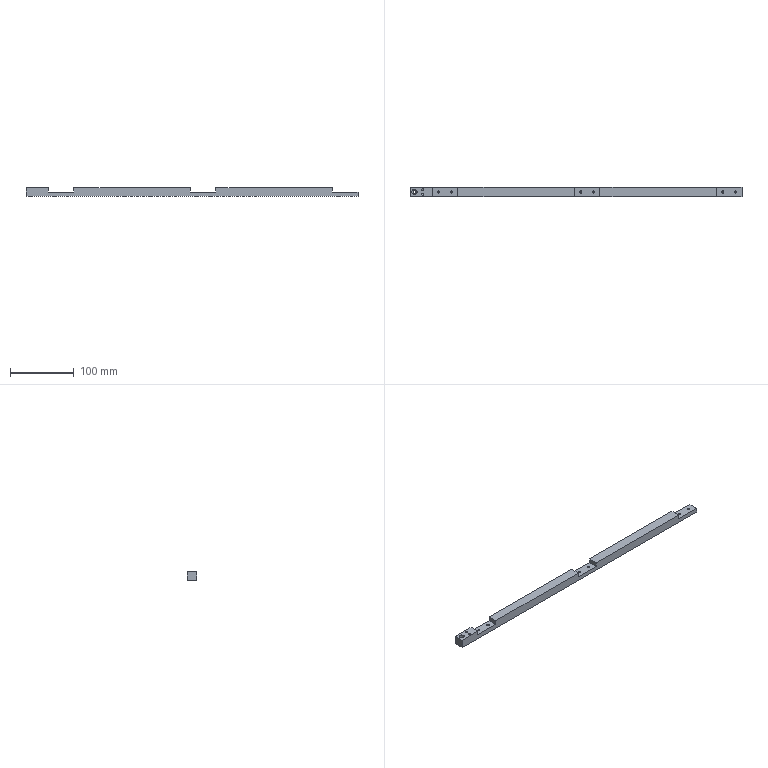CAM job | Mastercam | mm | 15 operations | part box 520 x 15 x 14
1. Facing | 24 - 100 平铣刀
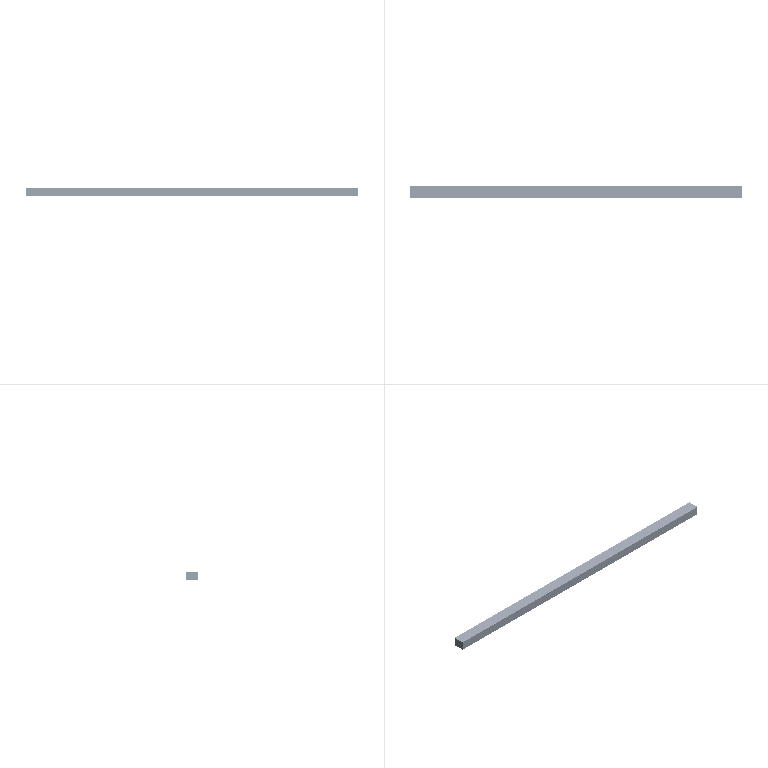2. Contour (Ramp) | 10 - 10 平铣刀
3. Contour (2D) | 10 - 10 平铣刀
4. Contour (2D chamfer) | 7 - 4 倒角刀
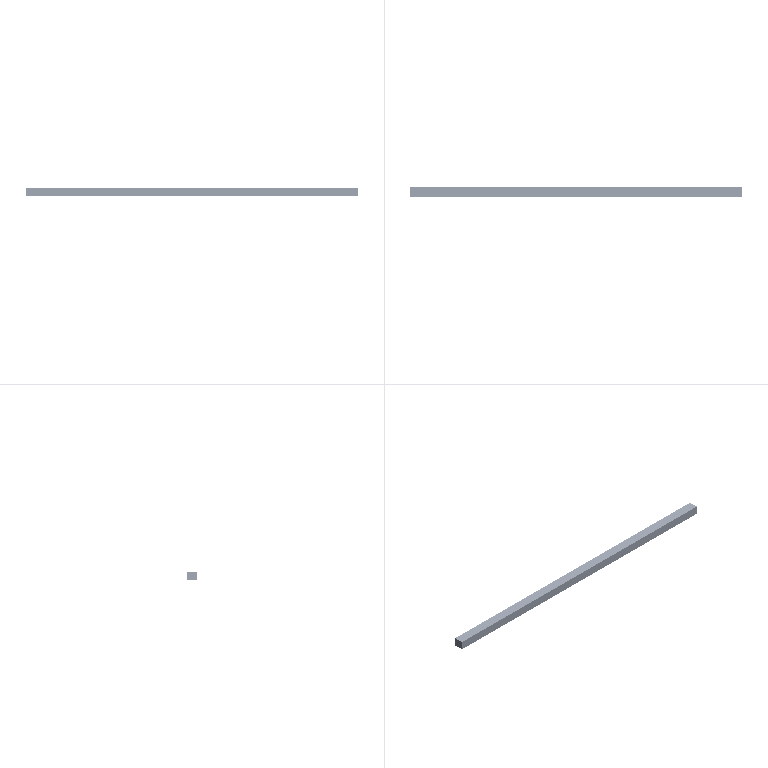5. Facing | 24 - 100 平铣刀
6. Contour (Ramp) | 10 - 10 平铣刀
7. Contour (2D) | 10 - 10 平铣刀
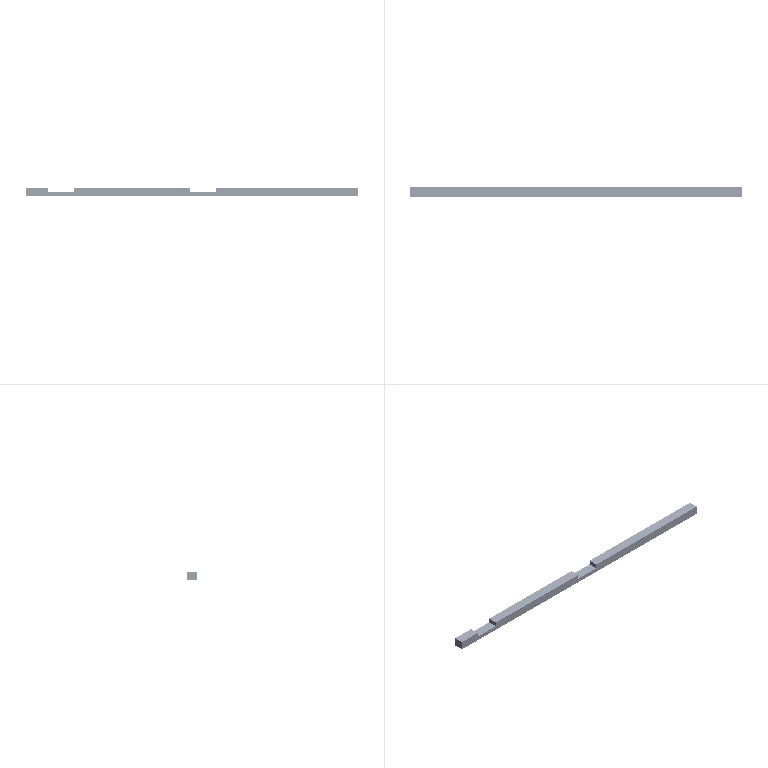8. Contour (Ramp) | 10 - 10 平铣刀
9. Contour (2D) | 10 - 10 平铣刀
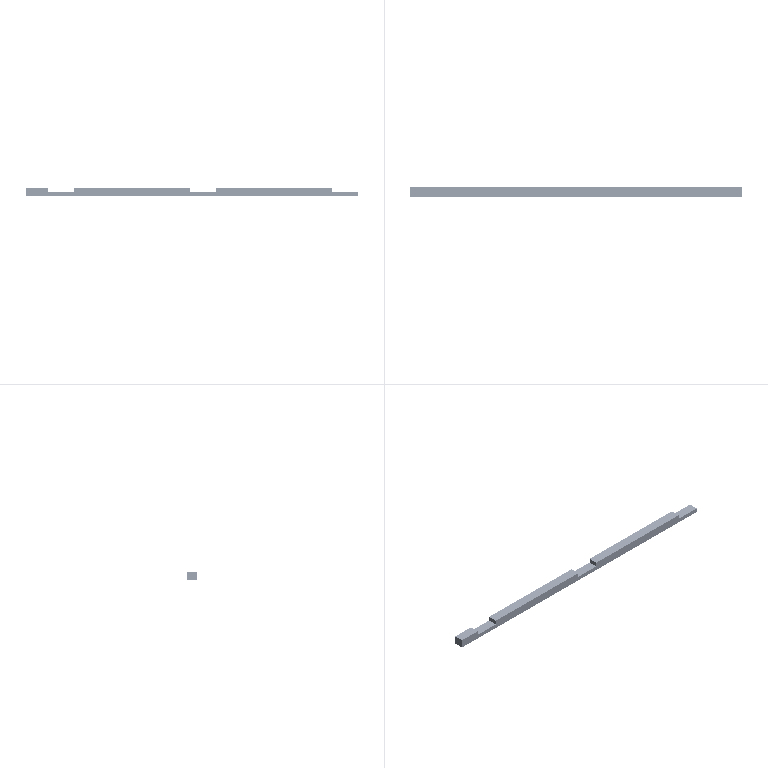10. Contour (Ramp) | 5 - 5 平铣刀
11. Contour (2D) | 5 - 5 平铣刀
12. Drill/Counterbore | 7 - 4 倒角刀
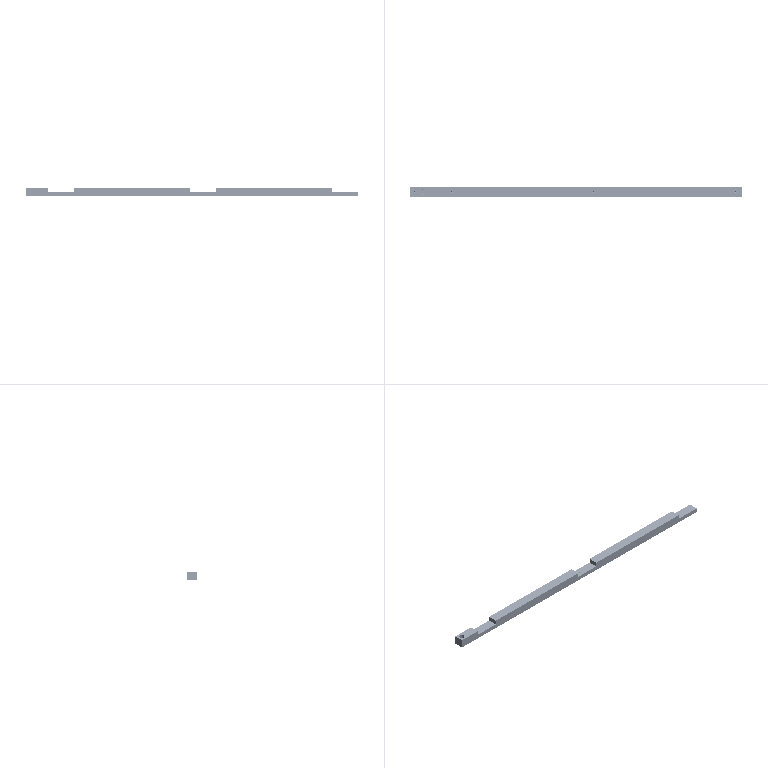13. Contour (2D chamfer) | 7 - 4 倒角刀
14. Contour (2D chamfer) | 7 - 4 倒角刀
15. Drill/Counterbore | 7 - 4 倒角刀